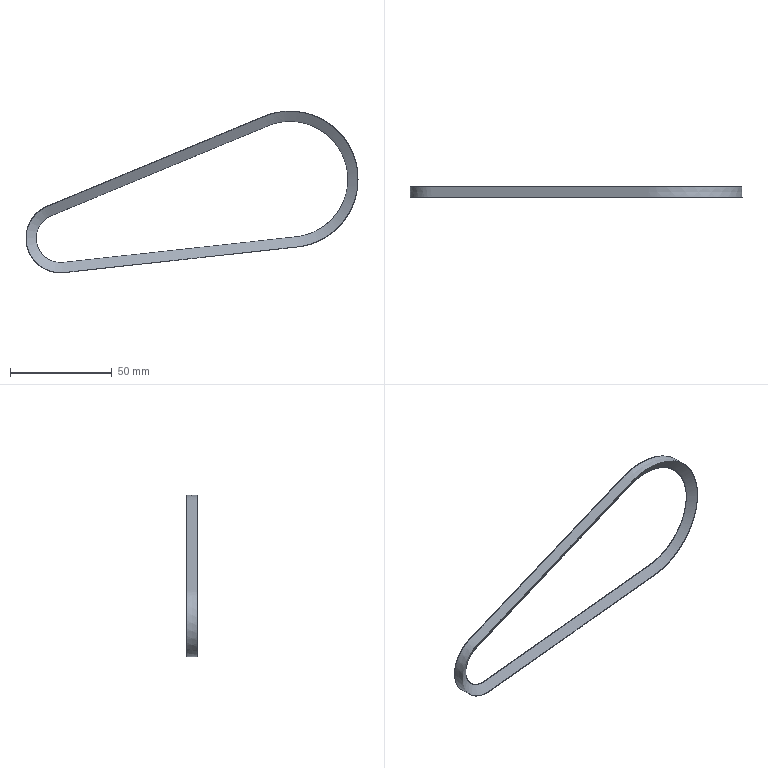Component | NX | BELT_2 | 1 solid | 1 faces | volume 4801 mm3 | spline 1